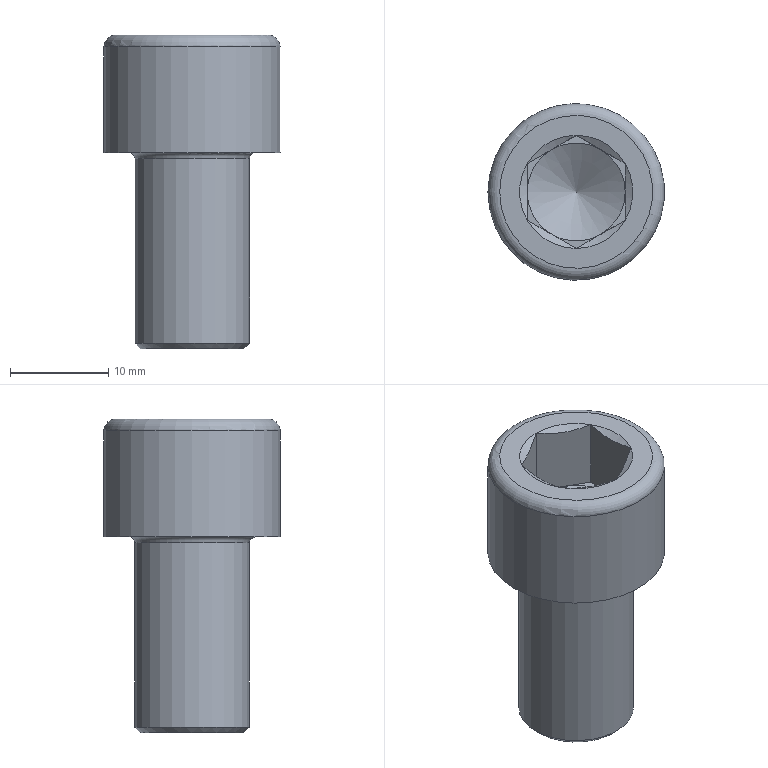Component | NX | GB-T70_1-2000_M12X20 | 1 solid | 27 faces | volume 4482 mm3 | plane 15 | cone 8 | cylinder 2 | torus 2 | commonest cylinder face diameters 11.701 x1 18 x1